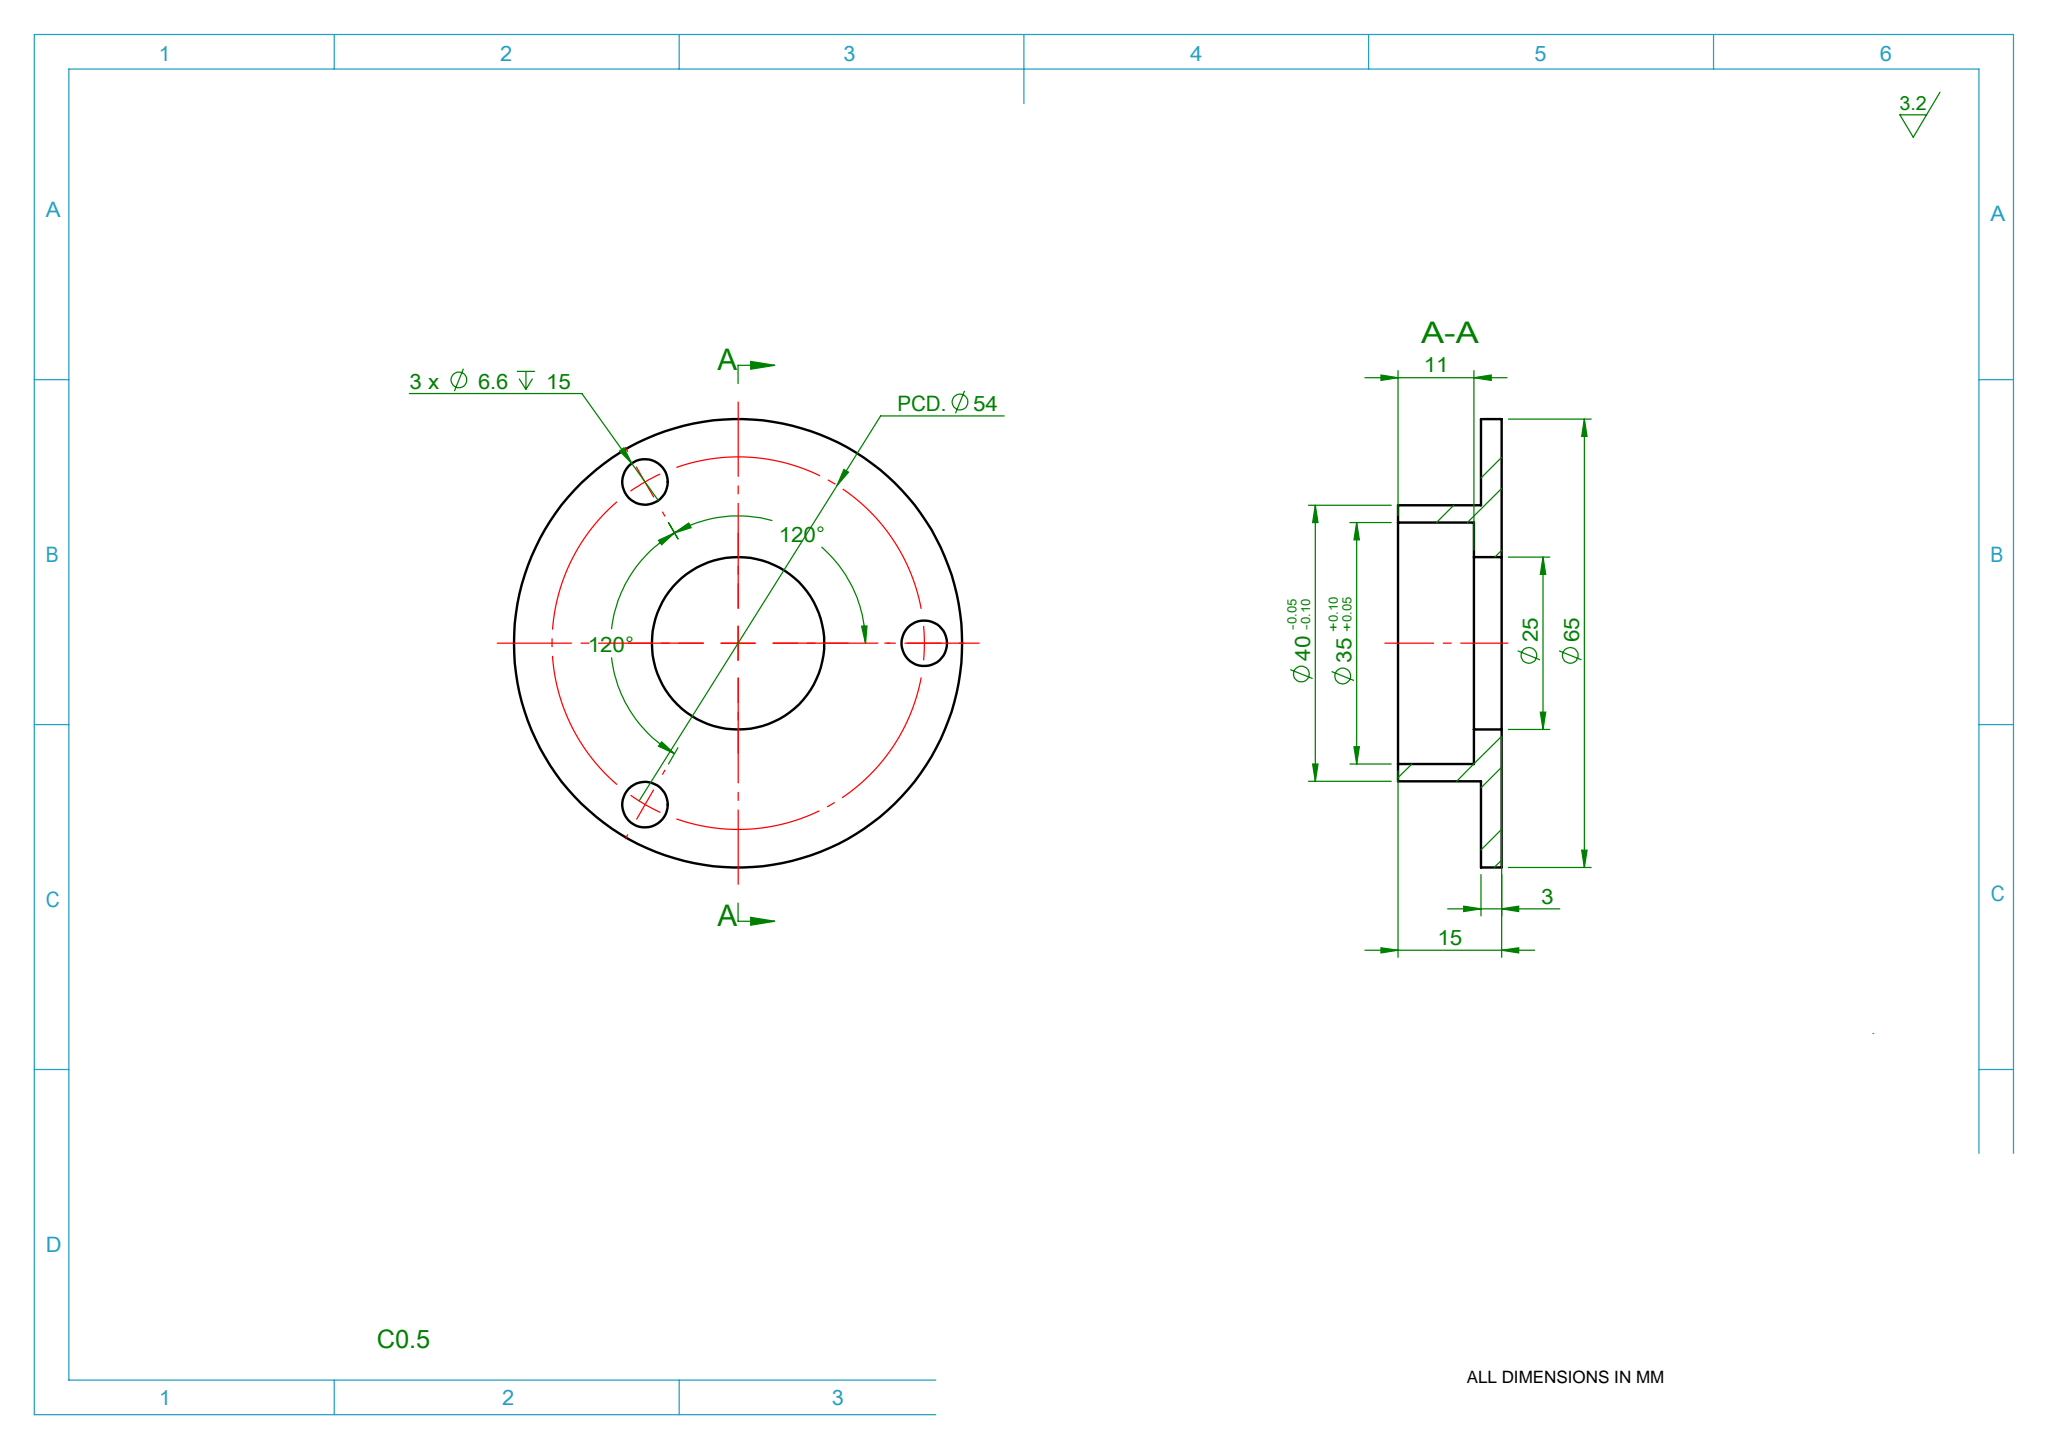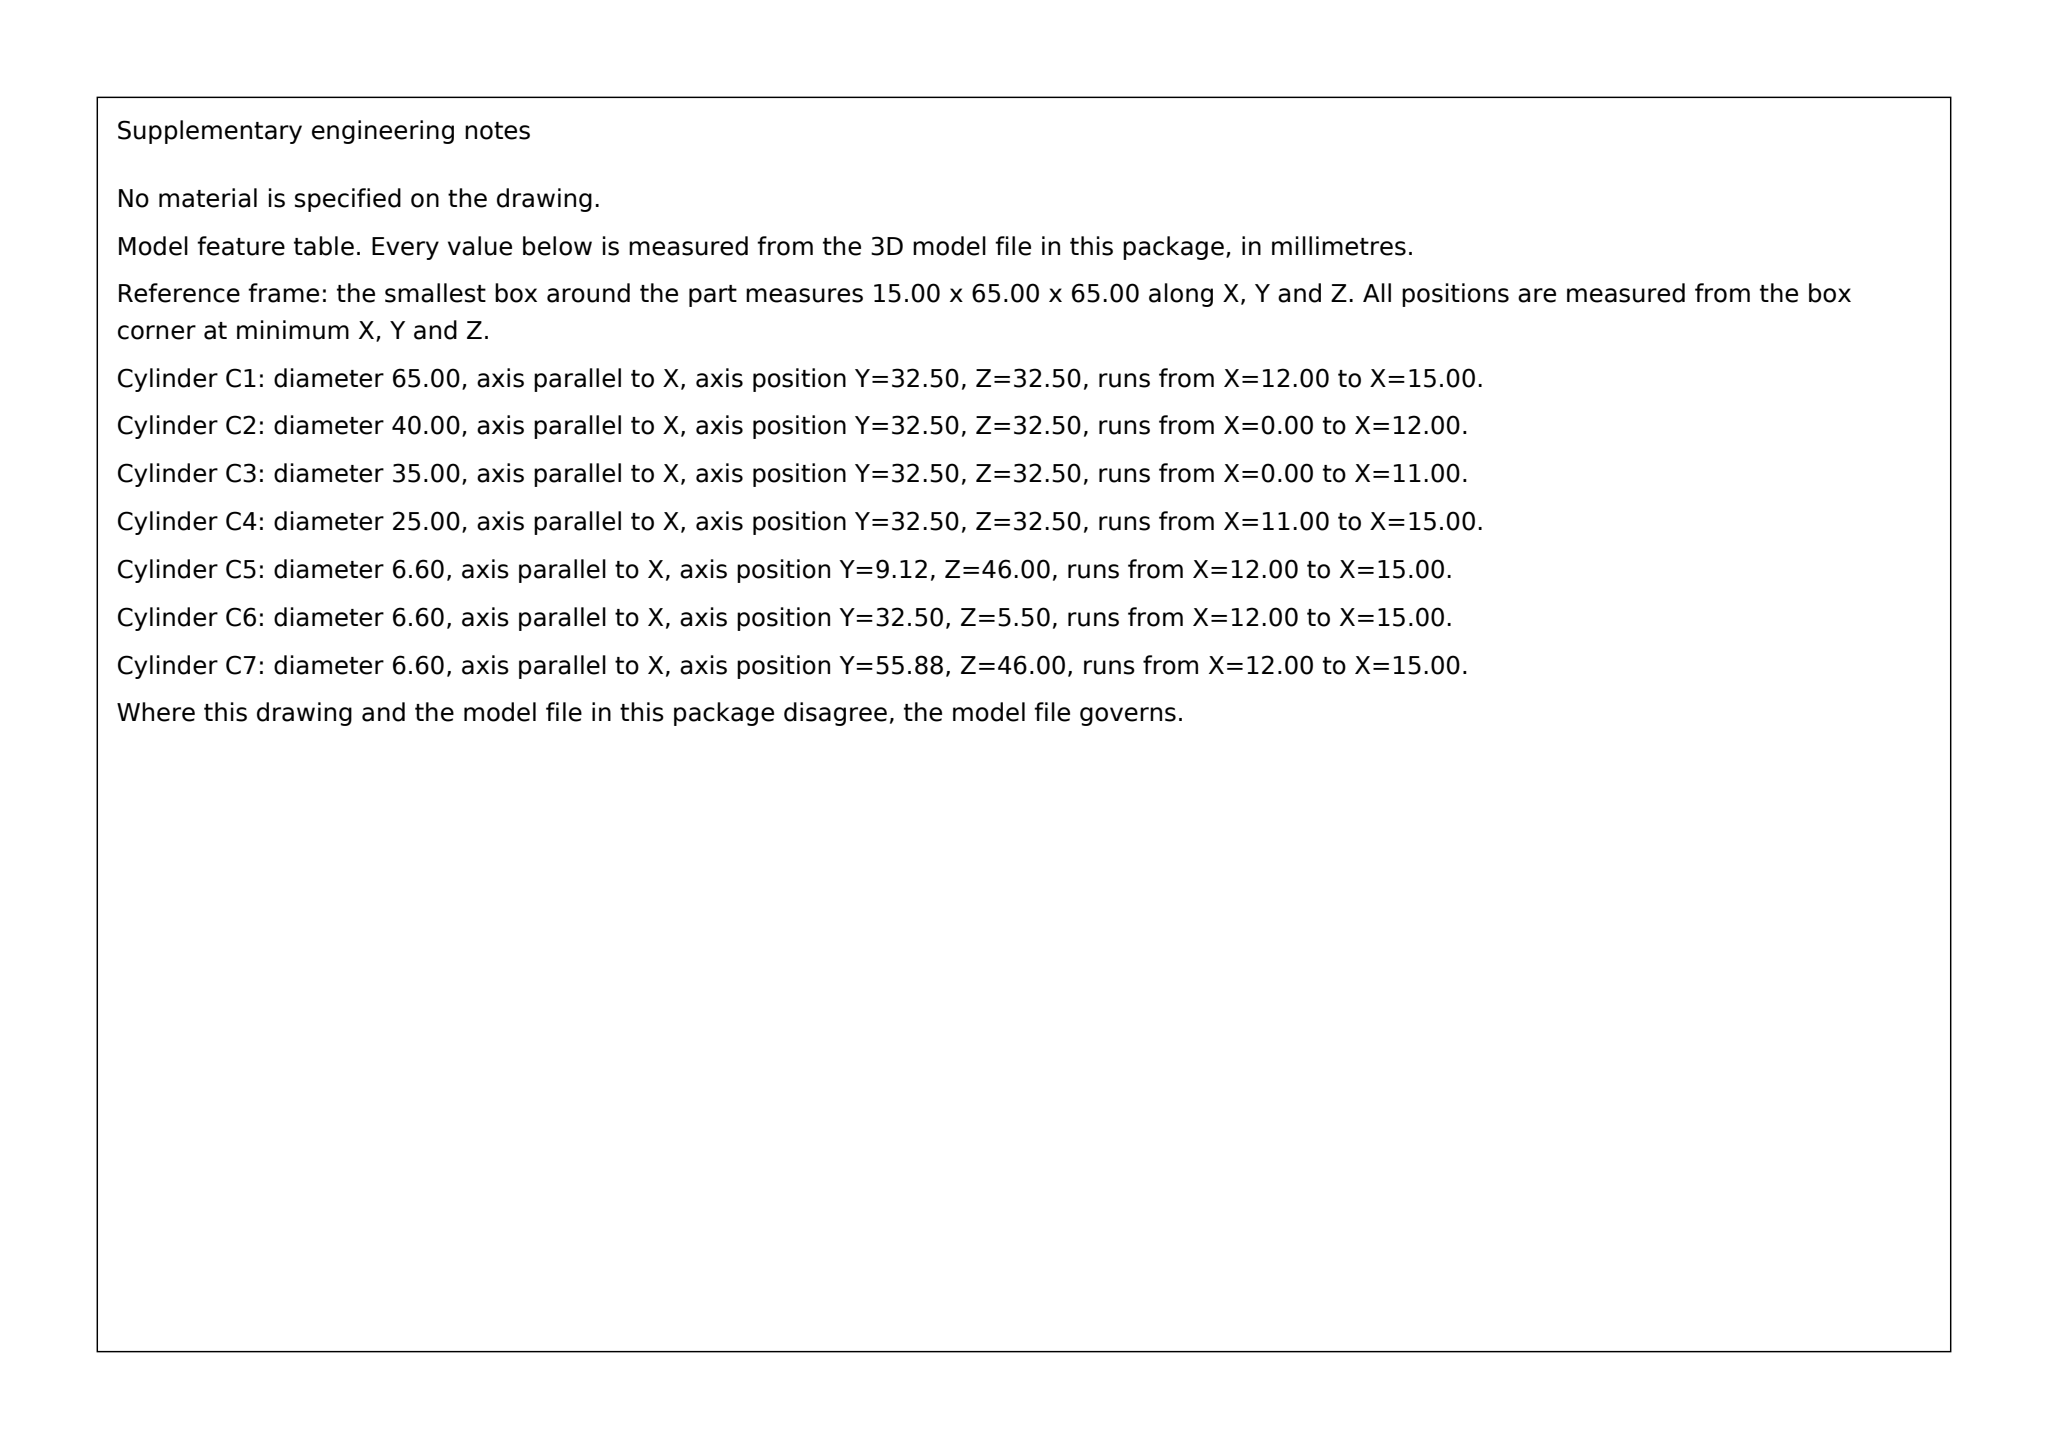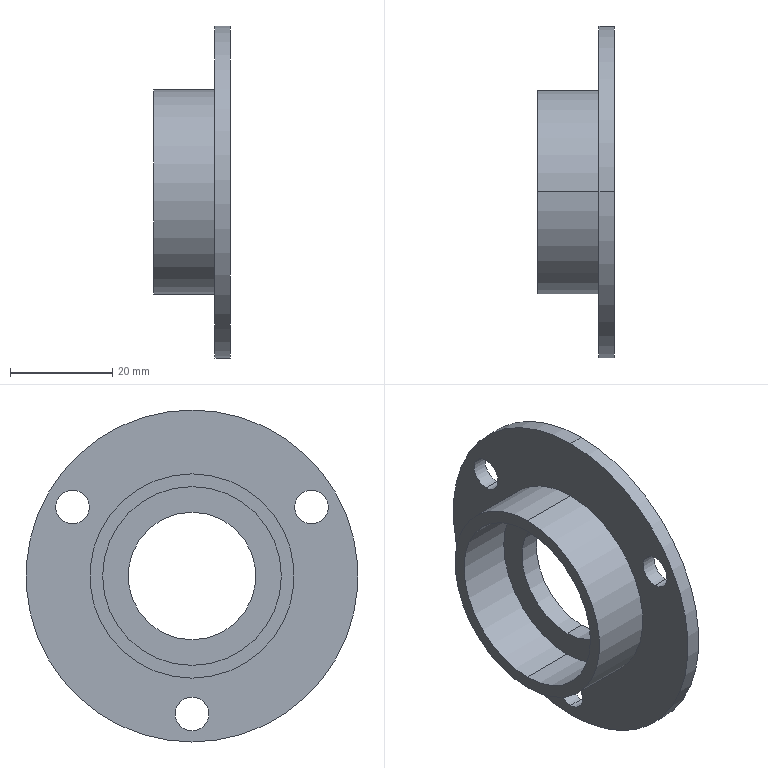Part | SolidWorks | mm | 1 solid | 18 faces | box 15 x 65 x 65 mm | volume 12180 mm3 | cylinder 14 | plane 4 | commonest cylinder face diameters 6.6 x6 35 x2 40 x2 65 x2 25 x2
build123d program:
from build123d import *

# Parameters (mm, degrees)
SKETCH1_R                = 32.5
SKETCH1_R_2              = 12.5
BOSS_EXTRUDE1_DEPTH      = 15
SKETCH2_R                = 32.5
SKETCH2_R_2              = 20
CUT_EXTRUDE1_DEPTH       = 30
SKETCH3_R                = 17.5
CUT_EXTRUDE2_DEPTH       = 11
M6_CLEARANCE_HOLE1_D     = 6.6
M6_CLEARANCE_HOLE1_DEPTH = 15
M6_CLEARANCE_HOLE1_TIP   = 1.983


with BuildPart() as part:
    # Sketch1 → Boss-Extrude1 (new body)
    with BuildSketch(Plane(origin=(0, 0, 0), x_dir=(0, 0, -1), z_dir=(1, 0, 0))):
        Circle(SKETCH1_R)
        Circle(SKETCH1_R_2, mode=Mode.SUBTRACT)
    extrude(amount=-BOSS_EXTRUDE1_DEPTH)

    # Sketch2 → Cut-Extrude1 (cut)
    with BuildSketch(Plane(origin=(-3, 0, 0), x_dir=(0, 0, -1), z_dir=(1, 0, 0))):
        Circle(SKETCH2_R)
        Circle(SKETCH2_R_2, mode=Mode.SUBTRACT)
    extrude(amount=-CUT_EXTRUDE1_DEPTH, mode=Mode.SUBTRACT)

    # Sketch3 → Cut-Extrude2 (cut)
    with BuildSketch(Plane.ZY.offset(15)):
        Circle(SKETCH3_R)
    extrude(amount=-CUT_EXTRUDE2_DEPTH, mode=Mode.SUBTRACT)

    # M6 Clearance Hole1
    with Locations(Plane(origin=(0, 0, 0), x_dir=(0, 0, -1), z_dir=(1, 0, 0))):
        with Locations((-13.5, 23.383), (-13.5, -23.383), (27, 0)):
            Hole(M6_CLEARANCE_HOLE1_D / 2, depth=M6_CLEARANCE_HOLE1_DEPTH)
            with Locations((0, 0, -(M6_CLEARANCE_HOLE1_DEPTH + M6_CLEARANCE_HOLE1_TIP / 2))):  # 118° drill point
                Cone(0, M6_CLEARANCE_HOLE1_D / 2, M6_CLEARANCE_HOLE1_TIP, mode=Mode.SUBTRACT)


solid = part.part
STEP:
#1=CARTESIAN_POINT('',(-3.,23.383,16.8));
#2=VERTEX_POINT('',#1);
#3=CARTESIAN_POINT('',(-3.,23.383,10.2));
#4=VERTEX_POINT('',#3);
#5=CARTESIAN_POINT('',(-3.,23.383,13.5));
#6=DIRECTION('',(1.,0.,0.));
#7=DIRECTION('',(0.,0.,-1.));
#8=AXIS2_PLACEMENT_3D('',#5,#6,#7);
#9=CIRCLE('',#8,3.3);
#10=EDGE_CURVE('',#2,#4,#9,.T.);
#11=ORIENTED_EDGE('',*,*,#10,.F.);
#12=CARTESIAN_POINT('',(-0.,23.383,16.8));
#13=VERTEX_POINT('',#12);
#14=CARTESIAN_POINT('',(0.,23.383,16.8));
#15=DIRECTION('',(1.,0.,0.));
#16=VECTOR('',#15,1000.);
#17=LINE('',#14,#16);
#18=EDGE_CURVE('',#2,#13,#17,.T.);
#19=ORIENTED_EDGE('',*,*,#18,.T.);
#20=CARTESIAN_POINT('',(-0.,23.383,10.2));
#21=VERTEX_POINT('',#20);
#22=CARTESIAN_POINT('',(-0.,23.383,13.5));
#23=DIRECTION('',(1.,0.,0.));
#24=DIRECTION('',(0.,0.,-1.));
#25=AXIS2_PLACEMENT_3D('',#22,#23,#24);
#26=CIRCLE('',#25,3.3);
#27=EDGE_CURVE('',#13,#21,#26,.T.);
#28=ORIENTED_EDGE('',*,*,#27,.T.);
#29=CARTESIAN_POINT('',(0.,23.383,10.2));
#30=DIRECTION('',(1.,0.,0.));
#31=VECTOR('',#30,1000.);
#32=LINE('',#29,#31);
#33=EDGE_CURVE('',#4,#21,#32,.T.);
#34=ORIENTED_EDGE('',*,*,#33,.F.);
#35=EDGE_LOOP('',(#11,#19,#28,#34));
#36=FACE_OUTER_BOUND('',#35,.T.);
#37=CARTESIAN_POINT('',(0.,23.383,13.5));
#38=DIRECTION('',(1.,0.,0.));
#39=DIRECTION('',(0.,0.,-1.));
#40=AXIS2_PLACEMENT_3D('',#37,#38,#39);
#41=CYLINDRICAL_SURFACE('',#40,3.3);
#42=ADVANCED_FACE('',(#36),#41,.F.);
#43=CARTESIAN_POINT('',(-3.,-23.383,16.8));
#44=VERTEX_POINT('',#43);
#45=CARTESIAN_POINT('',(-3.,-23.383,10.2));
#46=VERTEX_POINT('',#45);
#47=CARTESIAN_POINT('',(-3.,-23.383,13.5));
#48=DIRECTION('',(1.,0.,0.));
#49=DIRECTION('',(0.,0.,-1.));
#50=AXIS2_PLACEMENT_3D('',#47,#48,#49);
#51=CIRCLE('',#50,3.3);
#52=EDGE_CURVE('',#44,#46,#51,.T.);
#53=ORIENTED_EDGE('',*,*,#52,.F.);
#54=CARTESIAN_POINT('',(-0.,-23.383,16.8));
#55=VERTEX_POINT('',#54);
#56=CARTESIAN_POINT('',(0.,-23.383,16.8));
#57=DIRECTION('',(1.,0.,0.));
#58=VECTOR('',#57,1000.);
#59=LINE('',#56,#58);
#60=EDGE_CURVE('',#44,#55,#59,.T.);
#61=ORIENTED_EDGE('',*,*,#60,.T.);
#62=CARTESIAN_POINT('',(-0.,-23.383,10.2));
#63=VERTEX_POINT('',#62);
#64=CARTESIAN_POINT('',(-0.,-23.383,13.5));
#65=DIRECTION('',(1.,0.,0.));
#66=DIRECTION('',(0.,0.,-1.));
#67=AXIS2_PLACEMENT_3D('',#64,#65,#66);
#68=CIRCLE('',#67,3.3);
#69=EDGE_CURVE('',#55,#63,#68,.T.);
#70=ORIENTED_EDGE('',*,*,#69,.T.);
#71=CARTESIAN_POINT('',(0.,-23.383,10.2));
#72=DIRECTION('',(1.,0.,0.));
#73=VECTOR('',#72,1000.);
#74=LINE('',#71,#73);
#75=EDGE_CURVE('',#46,#63,#74,.T.);
#76=ORIENTED_EDGE('',*,*,#75,.F.);
#77=EDGE_LOOP('',(#53,#61,#70,#76));
#78=FACE_OUTER_BOUND('',#77,.T.);
#79=CARTESIAN_POINT('',(0.,-23.383,13.5));
#80=DIRECTION('',(1.,0.,0.));
#81=DIRECTION('',(0.,0.,-1.));
#82=AXIS2_PLACEMENT_3D('',#79,#80,#81);
#83=CYLINDRICAL_SURFACE('',#82,3.3);
#84=ADVANCED_FACE('',(#78),#83,.F.);
#85=CARTESIAN_POINT('',(-3.,0.,-23.7));
#86=VERTEX_POINT('',#85);
#87=CARTESIAN_POINT('',(-3.,0.,-30.3));
#88=VERTEX_POINT('',#87);
#89=CARTESIAN_POINT('',(-3.,0.,-27.));
#90=DIRECTION('',(1.,0.,0.));
#91=DIRECTION('',(0.,0.,-1.));
#92=AXIS2_PLACEMENT_3D('',#89,#90,#91);
#93=CIRCLE('',#92,3.3);
#94=EDGE_CURVE('',#86,#88,#93,.T.);
#95=ORIENTED_EDGE('',*,*,#94,.F.);
#96=CARTESIAN_POINT('',(-0.,0.,-23.7));
#97=VERTEX_POINT('',#96);
#98=CARTESIAN_POINT('',(0.,0.,-23.7));
#99=DIRECTION('',(1.,0.,0.));
#100=VECTOR('',#99,1000.);
#101=LINE('',#98,#100);
#102=EDGE_CURVE('',#86,#97,#101,.T.);
#103=ORIENTED_EDGE('',*,*,#102,.T.);
#104=CARTESIAN_POINT('',(-0.,0.,-30.3));
#105=VERTEX_POINT('',#104);
#106=CARTESIAN_POINT('',(-0.,0.,-27.));
#107=DIRECTION('',(1.,0.,0.));
#108=DIRECTION('',(0.,0.,-1.));
#109=AXIS2_PLACEMENT_3D('',#106,#107,#108);
#110=CIRCLE('',#109,3.3);
#111=EDGE_CURVE('',#97,#105,#110,.T.);
#112=ORIENTED_EDGE('',*,*,#111,.T.);
#113=CARTESIAN_POINT('',(0.,0.,-30.3));
#114=DIRECTION('',(1.,0.,0.));
#115=VECTOR('',#114,1000.);
#116=LINE('',#113,#115);
#117=EDGE_CURVE('',#88,#105,#116,.T.);
#118=ORIENTED_EDGE('',*,*,#117,.F.);
#119=EDGE_LOOP('',(#95,#103,#112,#118));
#120=FACE_OUTER_BOUND('',#119,.T.);
#121=CARTESIAN_POINT('',(0.,0.,-27.));
#122=DIRECTION('',(1.,0.,0.));
#123=DIRECTION('',(0.,0.,-1.));
#124=AXIS2_PLACEMENT_3D('',#121,#122,#123);
#125=CYLINDRICAL_SURFACE('',#124,3.3);
#126=ADVANCED_FACE('',(#120),#125,.F.);
#127=CARTESIAN_POINT('',(-4.,0.,-17.5));
#128=VERTEX_POINT('',#127);
#129=CARTESIAN_POINT('',(-4.,0.,17.5));
#130=VERTEX_POINT('',#129);
#131=CARTESIAN_POINT('',(-4.,0.,0.));
#132=DIRECTION('',(-1.,0.,0.));
#133=DIRECTION('',(0.,0.,1.));
#134=AXIS2_PLACEMENT_3D('',#131,#132,#133);
#135=CIRCLE('',#134,17.5);
#136=EDGE_CURVE('',#128,#130,#135,.T.);
#137=ORIENTED_EDGE('',*,*,#136,.F.);
#138=CARTESIAN_POINT('',(-15.,0.,-17.5));
#139=VERTEX_POINT('',#138);
#140=CARTESIAN_POINT('',(-4.,0.,-17.5));
#141=DIRECTION('',(-1.,0.,0.));
#142=VECTOR('',#141,1000.);
#143=LINE('',#140,#142);
#144=EDGE_CURVE('',#128,#139,#143,.T.);
#145=ORIENTED_EDGE('',*,*,#144,.T.);
#146=CARTESIAN_POINT('',(-15.,0.,17.5));
#147=VERTEX_POINT('',#146);
#148=CARTESIAN_POINT('',(-15.,0.,0.));
#149=DIRECTION('',(-1.,0.,0.));
#150=DIRECTION('',(0.,0.,1.));
#151=AXIS2_PLACEMENT_3D('',#148,#149,#150);
#152=CIRCLE('',#151,17.5);
#153=EDGE_CURVE('',#139,#147,#152,.T.);
#154=ORIENTED_EDGE('',*,*,#153,.T.);
#155=CARTESIAN_POINT('',(-4.,0.,17.5));
#156=DIRECTION('',(-1.,0.,0.));
#157=VECTOR('',#156,1000.);
#158=LINE('',#155,#157);
#159=EDGE_CURVE('',#130,#147,#158,.T.);
#160=ORIENTED_EDGE('',*,*,#159,.F.);
#161=EDGE_LOOP('',(#137,#145,#154,#160));
#162=FACE_OUTER_BOUND('',#161,.T.);
#163=CARTESIAN_POINT('',(-4.,0.,0.));
#164=DIRECTION('',(-1.,0.,0.));
#165=DIRECTION('',(0.,0.,1.));
#166=AXIS2_PLACEMENT_3D('',#163,#164,#165);
#167=CYLINDRICAL_SURFACE('',#166,17.5);
#168=ADVANCED_FACE('',(#162),#167,.F.);
#169=CARTESIAN_POINT('',(-15.,0.,-20.));
#170=VERTEX_POINT('',#169);
#171=CARTESIAN_POINT('',(-15.,0.,20.));
#172=VERTEX_POINT('',#171);
#173=CARTESIAN_POINT('',(-15.,0.,0.));
#174=DIRECTION('',(1.,0.,0.));
#175=DIRECTION('',(0.,0.,-1.));
#176=AXIS2_PLACEMENT_3D('',#173,#174,#175);
#177=CIRCLE('',#176,20.);
#178=EDGE_CURVE('',#170,#172,#177,.T.);
#179=ORIENTED_EDGE('',*,*,#178,.T.);
#180=CARTESIAN_POINT('',(-3.,0.,20.));
#181=VERTEX_POINT('',#180);
#182=CARTESIAN_POINT('',(-33.,0.,20.));
#183=DIRECTION('',(1.,0.,0.));
#184=VECTOR('',#183,1000.);
#185=LINE('',#182,#184);
#186=EDGE_CURVE('',#172,#181,#185,.T.);
#187=ORIENTED_EDGE('',*,*,#186,.T.);
#188=CARTESIAN_POINT('',(-3.,0.,-20.));
#189=VERTEX_POINT('',#188);
#190=CARTESIAN_POINT('',(-3.,0.,0.));
#191=DIRECTION('',(1.,0.,0.));
#192=DIRECTION('',(0.,0.,-1.));
#193=AXIS2_PLACEMENT_3D('',#190,#191,#192);
#194=CIRCLE('',#193,20.);
#195=EDGE_CURVE('',#189,#181,#194,.T.);
#196=ORIENTED_EDGE('',*,*,#195,.F.);
#197=CARTESIAN_POINT('',(-33.,0.,-20.));
#198=DIRECTION('',(1.,0.,0.));
#199=VECTOR('',#198,1000.);
#200=LINE('',#197,#199);
#201=EDGE_CURVE('',#170,#189,#200,.T.);
#202=ORIENTED_EDGE('',*,*,#201,.F.);
#203=EDGE_LOOP('',(#179,#187,#196,#202));
#204=FACE_OUTER_BOUND('',#203,.T.);
#205=CARTESIAN_POINT('',(-33.,0.,0.));
#206=DIRECTION('',(1.,0.,0.));
#207=DIRECTION('',(0.,0.,-1.));
#208=AXIS2_PLACEMENT_3D('',#205,#206,#207);
#209=CYLINDRICAL_SURFACE('',#208,20.);
#210=ADVANCED_FACE('',(#204),#209,.T.);
#211=CARTESIAN_POINT('',(-3.,0.,-32.5));
#212=VERTEX_POINT('',#211);
#213=CARTESIAN_POINT('',(-3.,0.,32.5));
#214=VERTEX_POINT('',#213);
#215=CARTESIAN_POINT('',(-3.,0.,0.));
#216=DIRECTION('',(1.,0.,0.));
#217=DIRECTION('',(0.,0.,-1.));
#218=AXIS2_PLACEMENT_3D('',#215,#216,#217);
#219=CIRCLE('',#218,32.5);
#220=EDGE_CURVE('',#212,#214,#219,.T.);
#221=ORIENTED_EDGE('',*,*,#220,.T.);
#222=CARTESIAN_POINT('',(0.,0.,32.5));
#223=VERTEX_POINT('',#222);
#224=CARTESIAN_POINT('',(-15.,0.,32.5));
#225=DIRECTION('',(1.,0.,0.));
#226=VECTOR('',#225,1000.);
#227=LINE('',#224,#226);
#228=EDGE_CURVE('',#214,#223,#227,.T.);
#229=ORIENTED_EDGE('',*,*,#228,.T.);
#230=CARTESIAN_POINT('',(0.,0.,-32.5));
#231=VERTEX_POINT('',#230);
#232=CARTESIAN_POINT('',(0.,0.,0.));
#233=DIRECTION('',(1.,0.,0.));
#234=DIRECTION('',(0.,0.,-1.));
#235=AXIS2_PLACEMENT_3D('',#232,#233,#234);
#236=CIRCLE('',#235,32.5);
#237=EDGE_CURVE('',#231,#223,#236,.T.);
#238=ORIENTED_EDGE('',*,*,#237,.F.);
#239=CARTESIAN_POINT('',(-15.,0.,-32.5));
#240=DIRECTION('',(1.,0.,0.));
#241=VECTOR('',#240,1000.);
#242=LINE('',#239,#241);
#243=EDGE_CURVE('',#212,#231,#242,.T.);
#244=ORIENTED_EDGE('',*,*,#243,.F.);
#245=EDGE_LOOP('',(#221,#229,#238,#244));
#246=FACE_OUTER_BOUND('',#245,.T.);
#247=CARTESIAN_POINT('',(-15.,0.,0.));
#248=DIRECTION('',(1.,0.,0.));
#249=DIRECTION('',(0.,0.,-1.));
#250=AXIS2_PLACEMENT_3D('',#247,#248,#249);
#251=CYLINDRICAL_SURFACE('',#250,32.5);
#252=ADVANCED_FACE('',(#246),#251,.T.);
#253=CARTESIAN_POINT('',(-4.,0.,12.5));
#254=VERTEX_POINT('',#253);
#255=CARTESIAN_POINT('',(-4.,0.,-12.5));
#256=VERTEX_POINT('',#255);
#257=CARTESIAN_POINT('',(-4.,0.,0.));
#258=DIRECTION('',(1.,0.,0.));
#259=DIRECTION('',(0.,0.,1.));
#260=AXIS2_PLACEMENT_3D('',#257,#258,#259);
#261=CIRCLE('',#260,12.5);
#262=EDGE_CURVE('',#254,#256,#261,.T.);
#263=ORIENTED_EDGE('',*,*,#262,.F.);
#264=CARTESIAN_POINT('',(0.,0.,12.5));
#265=VERTEX_POINT('',#264);
#266=CARTESIAN_POINT('',(-15.,0.,12.5));
#267=DIRECTION('',(1.,0.,0.));
#268=VECTOR('',#267,1000.);
#269=LINE('',#266,#268);
#270=EDGE_CURVE('',#254,#265,#269,.T.);
#271=ORIENTED_EDGE('',*,*,#270,.T.);
#272=CARTESIAN_POINT('',(0.,0.,-12.5));
#273=VERTEX_POINT('',#272);
#274=CARTESIAN_POINT('',(0.,0.,0.));
#275=DIRECTION('',(1.,0.,0.));
#276=DIRECTION('',(0.,0.,-1.));
#277=AXIS2_PLACEMENT_3D('',#274,#275,#276);
#278=CIRCLE('',#277,12.5);
#279=EDGE_CURVE('',#265,#273,#278,.T.);
#280=ORIENTED_EDGE('',*,*,#279,.T.);
#281=CARTESIAN_POINT('',(-15.,0.,-12.5));
#282=DIRECTION('',(1.,0.,0.));
#283=VECTOR('',#282,1000.);
#284=LINE('',#281,#283);
#285=EDGE_CURVE('',#256,#273,#284,.T.);
#286=ORIENTED_EDGE('',*,*,#285,.F.);
#287=EDGE_LOOP('',(#263,#271,#280,#286));
#288=FACE_OUTER_BOUND('',#287,.T.);
#289=CARTESIAN_POINT('',(-15.,0.,0.));
#290=DIRECTION('',(1.,0.,0.));
#291=DIRECTION('',(0.,0.,-1.));
#292=AXIS2_PLACEMENT_3D('',#289,#290,#291);
#293=CYLINDRICAL_SURFACE('',#292,12.5);
#294=ADVANCED_FACE('',(#288),#293,.F.);
#295=ORIENTED_EDGE('',*,*,#270,.F.);
#296=CARTESIAN_POINT('',(-4.,0.,0.));
#297=DIRECTION('',(1.,0.,0.));
#298=DIRECTION('',(0.,0.,1.));
#299=AXIS2_PLACEMENT_3D('',#296,#297,#298);
#300=CIRCLE('',#299,12.5);
#301=EDGE_CURVE('',#256,#254,#300,.T.);
#302=ORIENTED_EDGE('',*,*,#301,.F.);
#303=ORIENTED_EDGE('',*,*,#285,.T.);
#304=CARTESIAN_POINT('',(0.,0.,0.));
#305=DIRECTION('',(1.,0.,0.));
#306=DIRECTION('',(0.,0.,-1.));
#307=AXIS2_PLACEMENT_3D('',#304,#305,#306);
#308=CIRCLE('',#307,12.5);
#309=EDGE_CURVE('',#273,#265,#308,.T.);
#310=ORIENTED_EDGE('',*,*,#309,.T.);
#311=EDGE_LOOP('',(#295,#302,#303,#310));
#312=FACE_OUTER_BOUND('',#311,.T.);
#313=CARTESIAN_POINT('',(-15.,0.,0.));
#314=DIRECTION('',(1.,0.,0.));
#315=DIRECTION('',(0.,0.,-1.));
#316=AXIS2_PLACEMENT_3D('',#313,#314,#315);
#317=CYLINDRICAL_SURFACE('',#316,12.5);
#318=ADVANCED_FACE('',(#312),#317,.F.);
#319=CARTESIAN_POINT('',(-15.,0.,0.));
#320=DIRECTION('',(-1.,0.,0.));
#321=DIRECTION('',(0.,0.,1.));
#322=AXIS2_PLACEMENT_3D('',#319,#320,#321);
#323=CIRCLE('',#322,17.5);
#324=EDGE_CURVE('',#147,#139,#323,.T.);
#325=ORIENTED_EDGE('',*,*,#324,.F.);
#326=ORIENTED_EDGE('',*,*,#153,.F.);
#327=EDGE_LOOP('',(#325,#326));
#328=FACE_BOUND('',#327,.T.);
#329=ORIENTED_EDGE('',*,*,#178,.F.);
#330=CARTESIAN_POINT('',(-15.,0.,0.));
#331=DIRECTION('',(1.,0.,0.));
#332=DIRECTION('',(0.,0.,-1.));
#333=AXIS2_PLACEMENT_3D('',#330,#331,#332);
#334=CIRCLE('',#333,20.);
#335=EDGE_CURVE('',#172,#170,#334,.T.);
#336=ORIENTED_EDGE('',*,*,#335,.F.);
#337=EDGE_LOOP('',(#329,#336));
#338=FACE_OUTER_BOUND('',#337,.T.);
#339=CARTESIAN_POINT('',(-15.,0.,0.));
#340=DIRECTION('',(1.,0.,0.));
#341=DIRECTION('',(0.,0.,-1.));
#342=AXIS2_PLACEMENT_3D('',#339,#340,#341);
#343=PLANE('',#342);
#344=ADVANCED_FACE('',(#328,#338),#343,.F.);
#345=ORIENTED_EDGE('',*,*,#228,.F.);
#346=CARTESIAN_POINT('',(-3.,0.,0.));
#347=DIRECTION('',(1.,0.,0.));
#348=DIRECTION('',(0.,0.,-1.));
#349=AXIS2_PLACEMENT_3D('',#346,#347,#348);
#350=CIRCLE('',#349,32.5);
#351=EDGE_CURVE('',#214,#212,#350,.T.);
#352=ORIENTED_EDGE('',*,*,#351,.T.);
#353=ORIENTED_EDGE('',*,*,#243,.T.);
#354=CARTESIAN_POINT('',(0.,0.,0.));
#355=DIRECTION('',(1.,0.,0.));
#356=DIRECTION('',(0.,0.,-1.));
#357=AXIS2_PLACEMENT_3D('',#354,#355,#356);
#358=CIRCLE('',#357,32.5);
#359=EDGE_CURVE('',#223,#231,#358,.T.);
#360=ORIENTED_EDGE('',*,*,#359,.F.);
#361=EDGE_LOOP('',(#345,#352,#353,#360));
#362=FACE_OUTER_BOUND('',#361,.T.);
#363=CARTESIAN_POINT('',(-15.,0.,0.));
#364=DIRECTION('',(1.,0.,0.));
#365=DIRECTION('',(0.,0.,-1.));
#366=AXIS2_PLACEMENT_3D('',#363,#364,#365);
#367=CYLINDRICAL_SURFACE('',#366,32.5);
#368=ADVANCED_FACE('',(#362),#367,.T.);
#369=CARTESIAN_POINT('',(-0.,23.383,13.5));
#370=DIRECTION('',(1.,0.,0.));
#371=DIRECTION('',(0.,0.,-1.));
#372=AXIS2_PLACEMENT_3D('',#369,#370,#371);
#373=CIRCLE('',#372,3.3);
#374=EDGE_CURVE('',#21,#13,#373,.T.);
#375=ORIENTED_EDGE('',*,*,#374,.F.);
#376=ORIENTED_EDGE('',*,*,#27,.F.);
#377=EDGE_LOOP('',(#375,#376));
#378=FACE_BOUND('',#377,.T.);
#379=CARTESIAN_POINT('',(-0.,-23.383,13.5));
#380=DIRECTION('',(1.,0.,0.));
#381=DIRECTION('',(0.,0.,-1.));
#382=AXIS2_PLACEMENT_3D('',#379,#380,#381);
#383=CIRCLE('',#382,3.3);
#384=EDGE_CURVE('',#63,#55,#383,.T.);
#385=ORIENTED_EDGE('',*,*,#384,.F.);
#386=ORIENTED_EDGE('',*,*,#69,.F.);
#387=EDGE_LOOP('',(#385,#386));
#388=FACE_BOUND('',#387,.T.);
#389=CARTESIAN_POINT('',(-0.,0.,-27.));
#390=DIRECTION('',(1.,0.,0.));
#391=DIRECTION('',(0.,0.,-1.));
#392=AXIS2_PLACEMENT_3D('',#389,#390,#391);
#393=CIRCLE('',#392,3.3);
#394=EDGE_CURVE('',#105,#97,#393,.T.);
#395=ORIENTED_EDGE('',*,*,#394,.F.);
#396=ORIENTED_EDGE('',*,*,#111,.F.);
#397=EDGE_LOOP('',(#395,#396));
#398=FACE_BOUND('',#397,.T.);
#399=ORIENTED_EDGE('',*,*,#309,.F.);
#400=ORIENTED_EDGE('',*,*,#279,.F.);
#401=EDGE_LOOP('',(#399,#400));
#402=FACE_BOUND('',#401,.T.);
#403=ORIENTED_EDGE('',*,*,#237,.T.);
#404=ORIENTED_EDGE('',*,*,#359,.T.);
#405=EDGE_LOOP('',(#403,#404));
#406=FACE_OUTER_BOUND('',#405,.T.);
#407=CARTESIAN_POINT('',(0.,0.,0.));
#408=DIRECTION('',(1.,0.,0.));
#409=DIRECTION('',(0.,0.,-1.));
#410=AXIS2_PLACEMENT_3D('',#407,#408,#409);
#411=PLANE('',#410);
#412=ADVANCED_FACE('',(#378,#388,#398,#402,#406),#411,.T.);
#413=ORIENTED_EDGE('',*,*,#186,.F.);
#414=ORIENTED_EDGE('',*,*,#335,.T.);
#415=ORIENTED_EDGE('',*,*,#201,.T.);
#416=CARTESIAN_POINT('',(-3.,0.,0.));
#417=DIRECTION('',(1.,0.,0.));
#418=DIRECTION('',(0.,0.,-1.));
#419=AXIS2_PLACEMENT_3D('',#416,#417,#418);
#420=CIRCLE('',#419,20.);
#421=EDGE_CURVE('',#181,#189,#420,.T.);
#422=ORIENTED_EDGE('',*,*,#421,.F.);
#423=EDGE_LOOP('',(#413,#414,#415,#422));
#424=FACE_OUTER_BOUND('',#423,.T.);
#425=CARTESIAN_POINT('',(-33.,0.,0.));
#426=DIRECTION('',(1.,0.,0.));
#427=DIRECTION('',(0.,0.,-1.));
#428=AXIS2_PLACEMENT_3D('',#425,#426,#427);
#429=CYLINDRICAL_SURFACE('',#428,20.);
#430=ADVANCED_FACE('',(#424),#429,.T.);
#431=CARTESIAN_POINT('',(-3.,23.383,13.5));
#432=DIRECTION('',(1.,0.,0.));
#433=DIRECTION('',(0.,0.,-1.));
#434=AXIS2_PLACEMENT_3D('',#431,#432,#433);
#435=CIRCLE('',#434,3.3);
#436=EDGE_CURVE('',#4,#2,#435,.T.);
#437=ORIENTED_EDGE('',*,*,#436,.T.);
#438=ORIENTED_EDGE('',*,*,#10,.T.);
#439=EDGE_LOOP('',(#437,#438));
#440=FACE_BOUND('',#439,.T.);
#441=CARTESIAN_POINT('',(-3.,-23.383,13.5));
#442=DIRECTION('',(1.,0.,0.));
#443=DIRECTION('',(0.,0.,-1.));
#444=AXIS2_PLACEMENT_3D('',#441,#442,#443);
#445=CIRCLE('',#444,3.3);
#446=EDGE_CURVE('',#46,#44,#445,.T.);
#447=ORIENTED_EDGE('',*,*,#446,.T.);
#448=ORIENTED_EDGE('',*,*,#52,.T.);
#449=EDGE_LOOP('',(#447,#448));
#450=FACE_BOUND('',#449,.T.);
#451=CARTESIAN_POINT('',(-3.,0.,-27.));
#452=DIRECTION('',(1.,0.,0.));
#453=DIRECTION('',(0.,0.,-1.));
#454=AXIS2_PLACEMENT_3D('',#451,#452,#453);
#455=CIRCLE('',#454,3.3);
#456=EDGE_CURVE('',#88,#86,#455,.T.);
#457=ORIENTED_EDGE('',*,*,#456,.T.);
#458=ORIENTED_EDGE('',*,*,#94,.T.);
#459=EDGE_LOOP('',(#457,#458));
#460=FACE_BOUND('',#459,.T.);
#461=ORIENTED_EDGE('',*,*,#195,.T.);
#462=ORIENTED_EDGE('',*,*,#421,.T.);
#463=EDGE_LOOP('',(#461,#462));
#464=FACE_BOUND('',#463,.T.);
#465=ORIENTED_EDGE('',*,*,#220,.F.);
#466=ORIENTED_EDGE('',*,*,#351,.F.);
#467=EDGE_LOOP('',(#465,#466));
#468=FACE_OUTER_BOUND('',#467,.T.);
#469=CARTESIAN_POINT('',(-3.,0.,0.));
#470=DIRECTION('',(1.,0.,0.));
#471=DIRECTION('',(0.,0.,-1.));
#472=AXIS2_PLACEMENT_3D('',#469,#470,#471);
#473=PLANE('',#472);
#474=ADVANCED_FACE('',(#440,#450,#460,#464,#468),#473,.F.);
#475=CARTESIAN_POINT('',(-4.,0.,0.));
#476=DIRECTION('',(-1.,0.,0.));
#477=DIRECTION('',(0.,0.,1.));
#478=AXIS2_PLACEMENT_3D('',#475,#476,#477);
#479=CIRCLE('',#478,17.5);
#480=EDGE_CURVE('',#130,#128,#479,.T.);
#481=ORIENTED_EDGE('',*,*,#480,.T.);
#482=ORIENTED_EDGE('',*,*,#136,.T.);
#483=EDGE_LOOP('',(#481,#482));
#484=FACE_OUTER_BOUND('',#483,.T.);
#485=ORIENTED_EDGE('',*,*,#301,.T.);
#486=ORIENTED_EDGE('',*,*,#262,.T.);
#487=EDGE_LOOP('',(#485,#486));
#488=FACE_BOUND('',#487,.T.);
#489=CARTESIAN_POINT('',(-4.,0.,0.));
#490=DIRECTION('',(-1.,0.,0.));
#491=DIRECTION('',(0.,0.,1.));
#492=AXIS2_PLACEMENT_3D('',#489,#490,#491);
#493=PLANE('',#492);
#494=ADVANCED_FACE('',(#484,#488),#493,.T.);
#495=ORIENTED_EDGE('',*,*,#144,.F.);
#496=ORIENTED_EDGE('',*,*,#480,.F.);
#497=ORIENTED_EDGE('',*,*,#159,.T.);
#498=ORIENTED_EDGE('',*,*,#324,.T.);
#499=EDGE_LOOP('',(#495,#496,#497,#498));
#500=FACE_OUTER_BOUND('',#499,.T.);
#501=CARTESIAN_POINT('',(-4.,0.,0.));
#502=DIRECTION('',(-1.,0.,0.));
#503=DIRECTION('',(0.,0.,1.));
#504=AXIS2_PLACEMENT_3D('',#501,#502,#503);
#505=CYLINDRICAL_SURFACE('',#504,17.5);
#506=ADVANCED_FACE('',(#500),#505,.F.);
#507=ORIENTED_EDGE('',*,*,#102,.F.);
#508=ORIENTED_EDGE('',*,*,#456,.F.);
#509=ORIENTED_EDGE('',*,*,#117,.T.);
#510=ORIENTED_EDGE('',*,*,#394,.T.);
#511=EDGE_LOOP('',(#507,#508,#509,#510));
#512=FACE_OUTER_BOUND('',#511,.T.);
#513=CARTESIAN_POINT('',(0.,0.,-27.));
#514=DIRECTION('',(1.,0.,0.));
#515=DIRECTION('',(0.,0.,-1.));
#516=AXIS2_PLACEMENT_3D('',#513,#514,#515);
#517=CYLINDRICAL_SURFACE('',#516,3.3);
#518=ADVANCED_FACE('',(#512),#517,.F.);
#519=ORIENTED_EDGE('',*,*,#60,.F.);
#520=ORIENTED_EDGE('',*,*,#446,.F.);
#521=ORIENTED_EDGE('',*,*,#75,.T.);
#522=ORIENTED_EDGE('',*,*,#384,.T.);
#523=EDGE_LOOP('',(#519,#520,#521,#522));
#524=FACE_OUTER_BOUND('',#523,.T.);
#525=CARTESIAN_POINT('',(0.,-23.383,13.5));
#526=DIRECTION('',(1.,0.,0.));
#527=DIRECTION('',(0.,0.,-1.));
#528=AXIS2_PLACEMENT_3D('',#525,#526,#527);
#529=CYLINDRICAL_SURFACE('',#528,3.3);
#530=ADVANCED_FACE('',(#524),#529,.F.);
#531=ORIENTED_EDGE('',*,*,#18,.F.);
#532=ORIENTED_EDGE('',*,*,#436,.F.);
#533=ORIENTED_EDGE('',*,*,#33,.T.);
#534=ORIENTED_EDGE('',*,*,#374,.T.);
#535=EDGE_LOOP('',(#531,#532,#533,#534));
#536=FACE_OUTER_BOUND('',#535,.T.);
#537=CARTESIAN_POINT('',(0.,23.383,13.5));
#538=DIRECTION('',(1.,0.,0.));
#539=DIRECTION('',(0.,0.,-1.));
#540=AXIS2_PLACEMENT_3D('',#537,#538,#539);
#541=CYLINDRICAL_SURFACE('',#540,3.3);
#542=ADVANCED_FACE('',(#536),#541,.F.);
#543=CLOSED_SHELL('',(#42,#84,#126,#168,#210,#252,#294,#318,#344,#368,#412,#430,#474,#494,#506,#518,#530,#542));
#544=MANIFOLD_SOLID_BREP('',#543);
#545=CARTESIAN_POINT('',(0.,0.,0.));
#546=DIRECTION('',(0.,0.,1.));
#547=DIRECTION('',(1.,0.,0.));
#548=AXIS2_PLACEMENT_3D('',#545,#546,#547);
#549=(LENGTH_UNIT()NAMED_UNIT(*)SI_UNIT(.MILLI.,.METRE.));
#550=UNCERTAINTY_MEASURE_WITH_UNIT(LENGTH_MEASURE(0.00001),#549,'','');
#551=(NAMED_UNIT(*)PLANE_ANGLE_UNIT()SI_UNIT($,.RADIAN.));
#552=(NAMED_UNIT(*)SI_UNIT($,.STERADIAN.)SOLID_ANGLE_UNIT());
#553=(GEOMETRIC_REPRESENTATION_CONTEXT(3)GLOBAL_UNCERTAINTY_ASSIGNED_CONTEXT((#550))GLOBAL_UNIT_ASSIGNED_CONTEXT((#549,#551,#552))REPRESENTATION_CONTEXT('',''));
#554=ADVANCED_BREP_SHAPE_REPRESENTATION('',(#544,#548),#553);